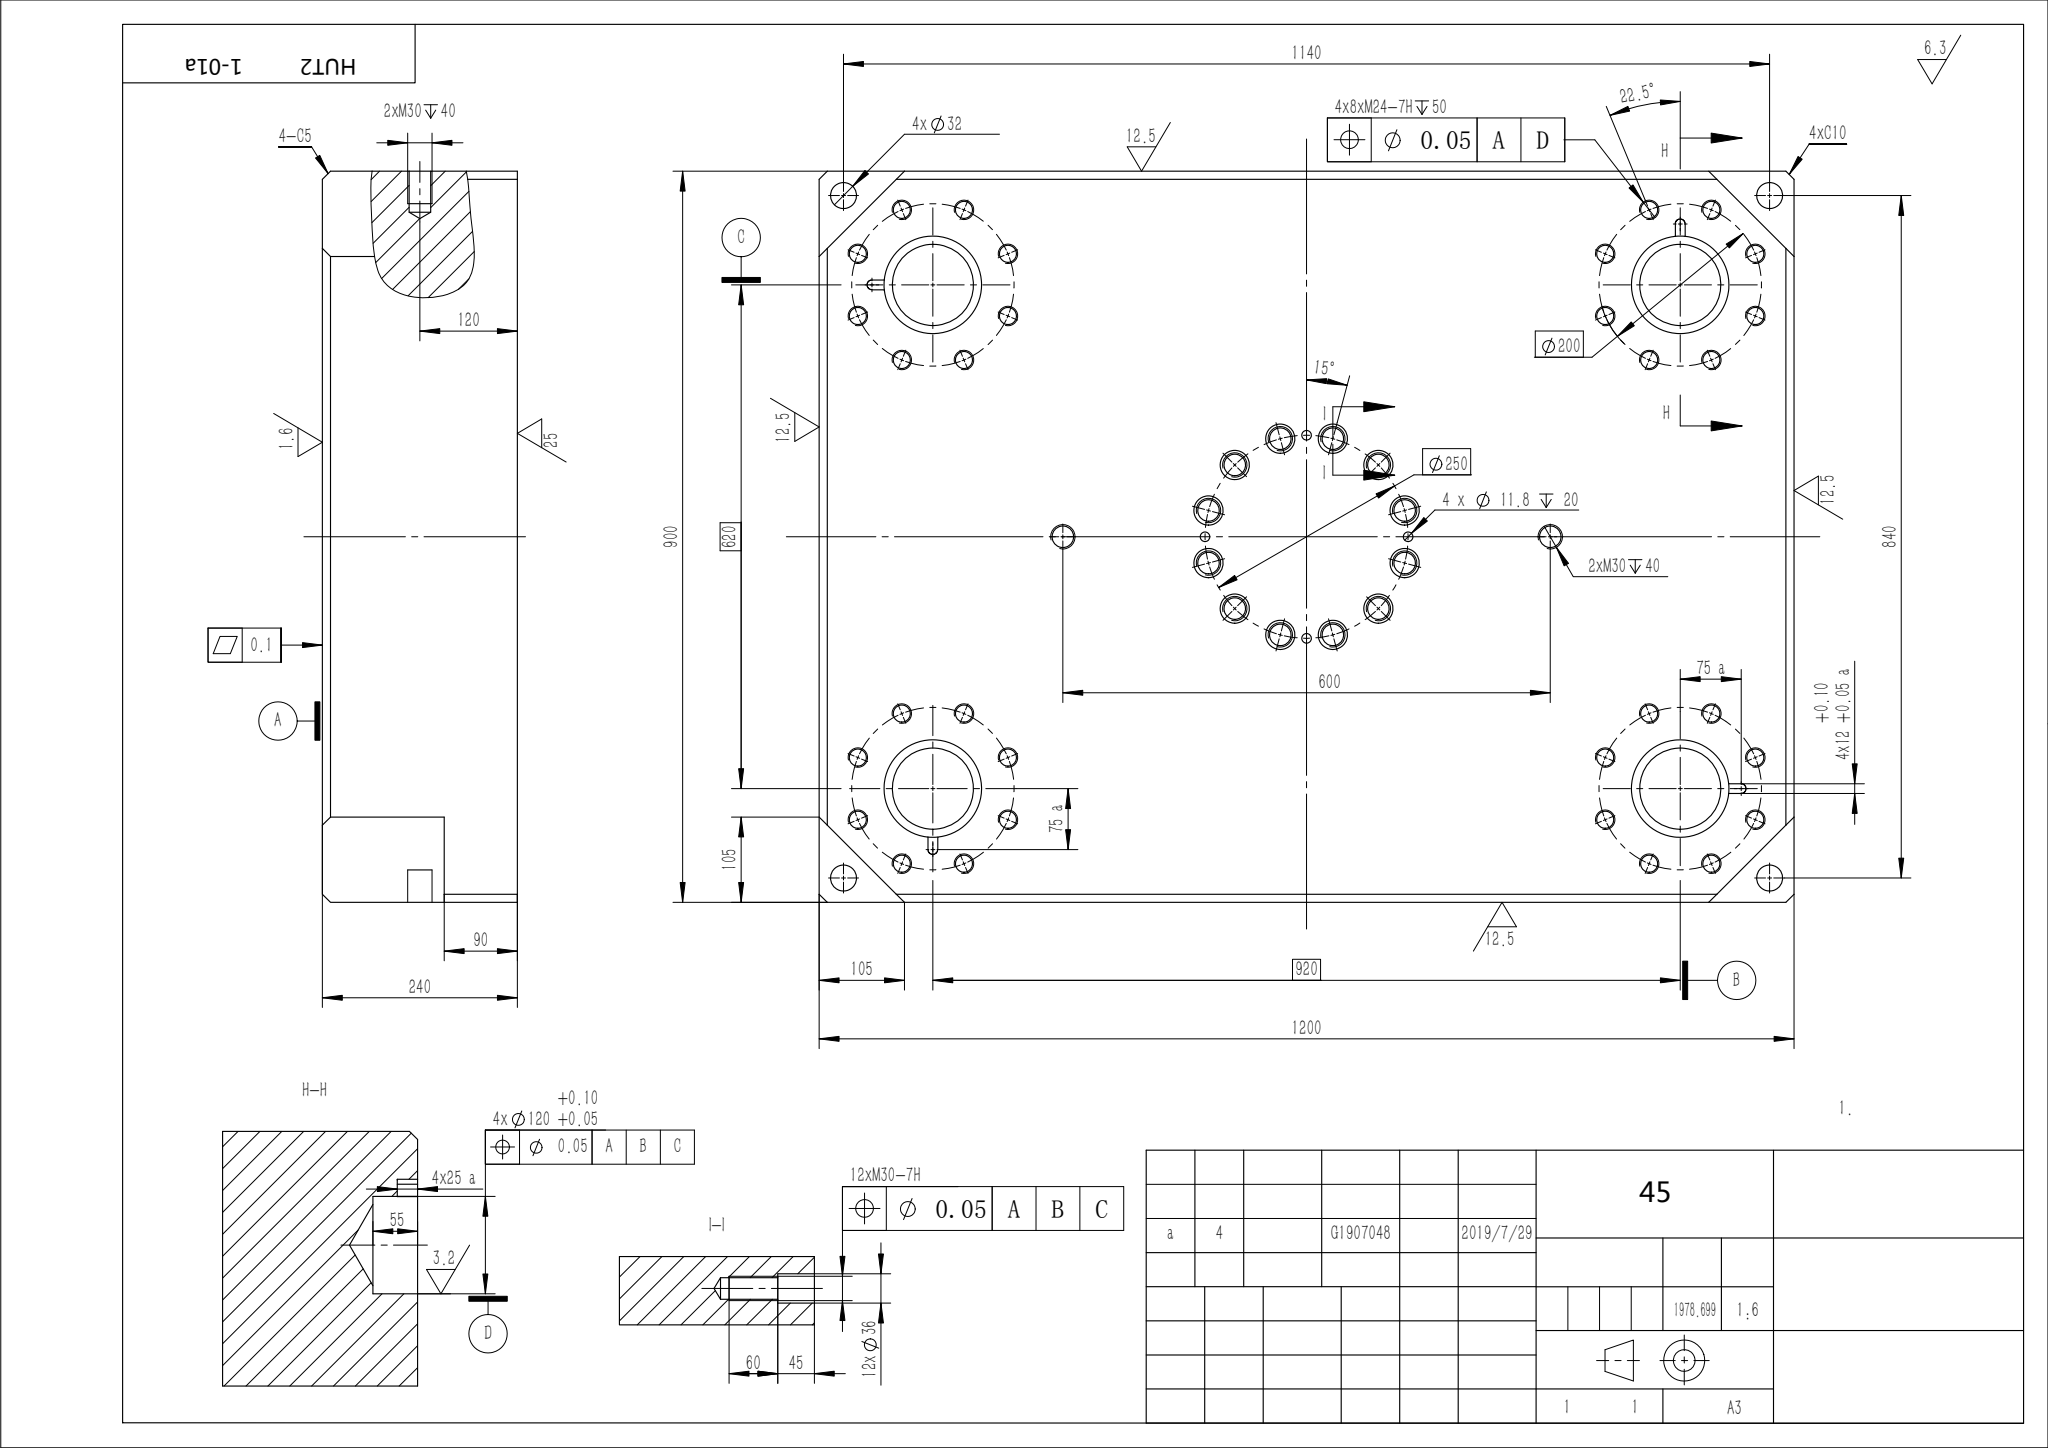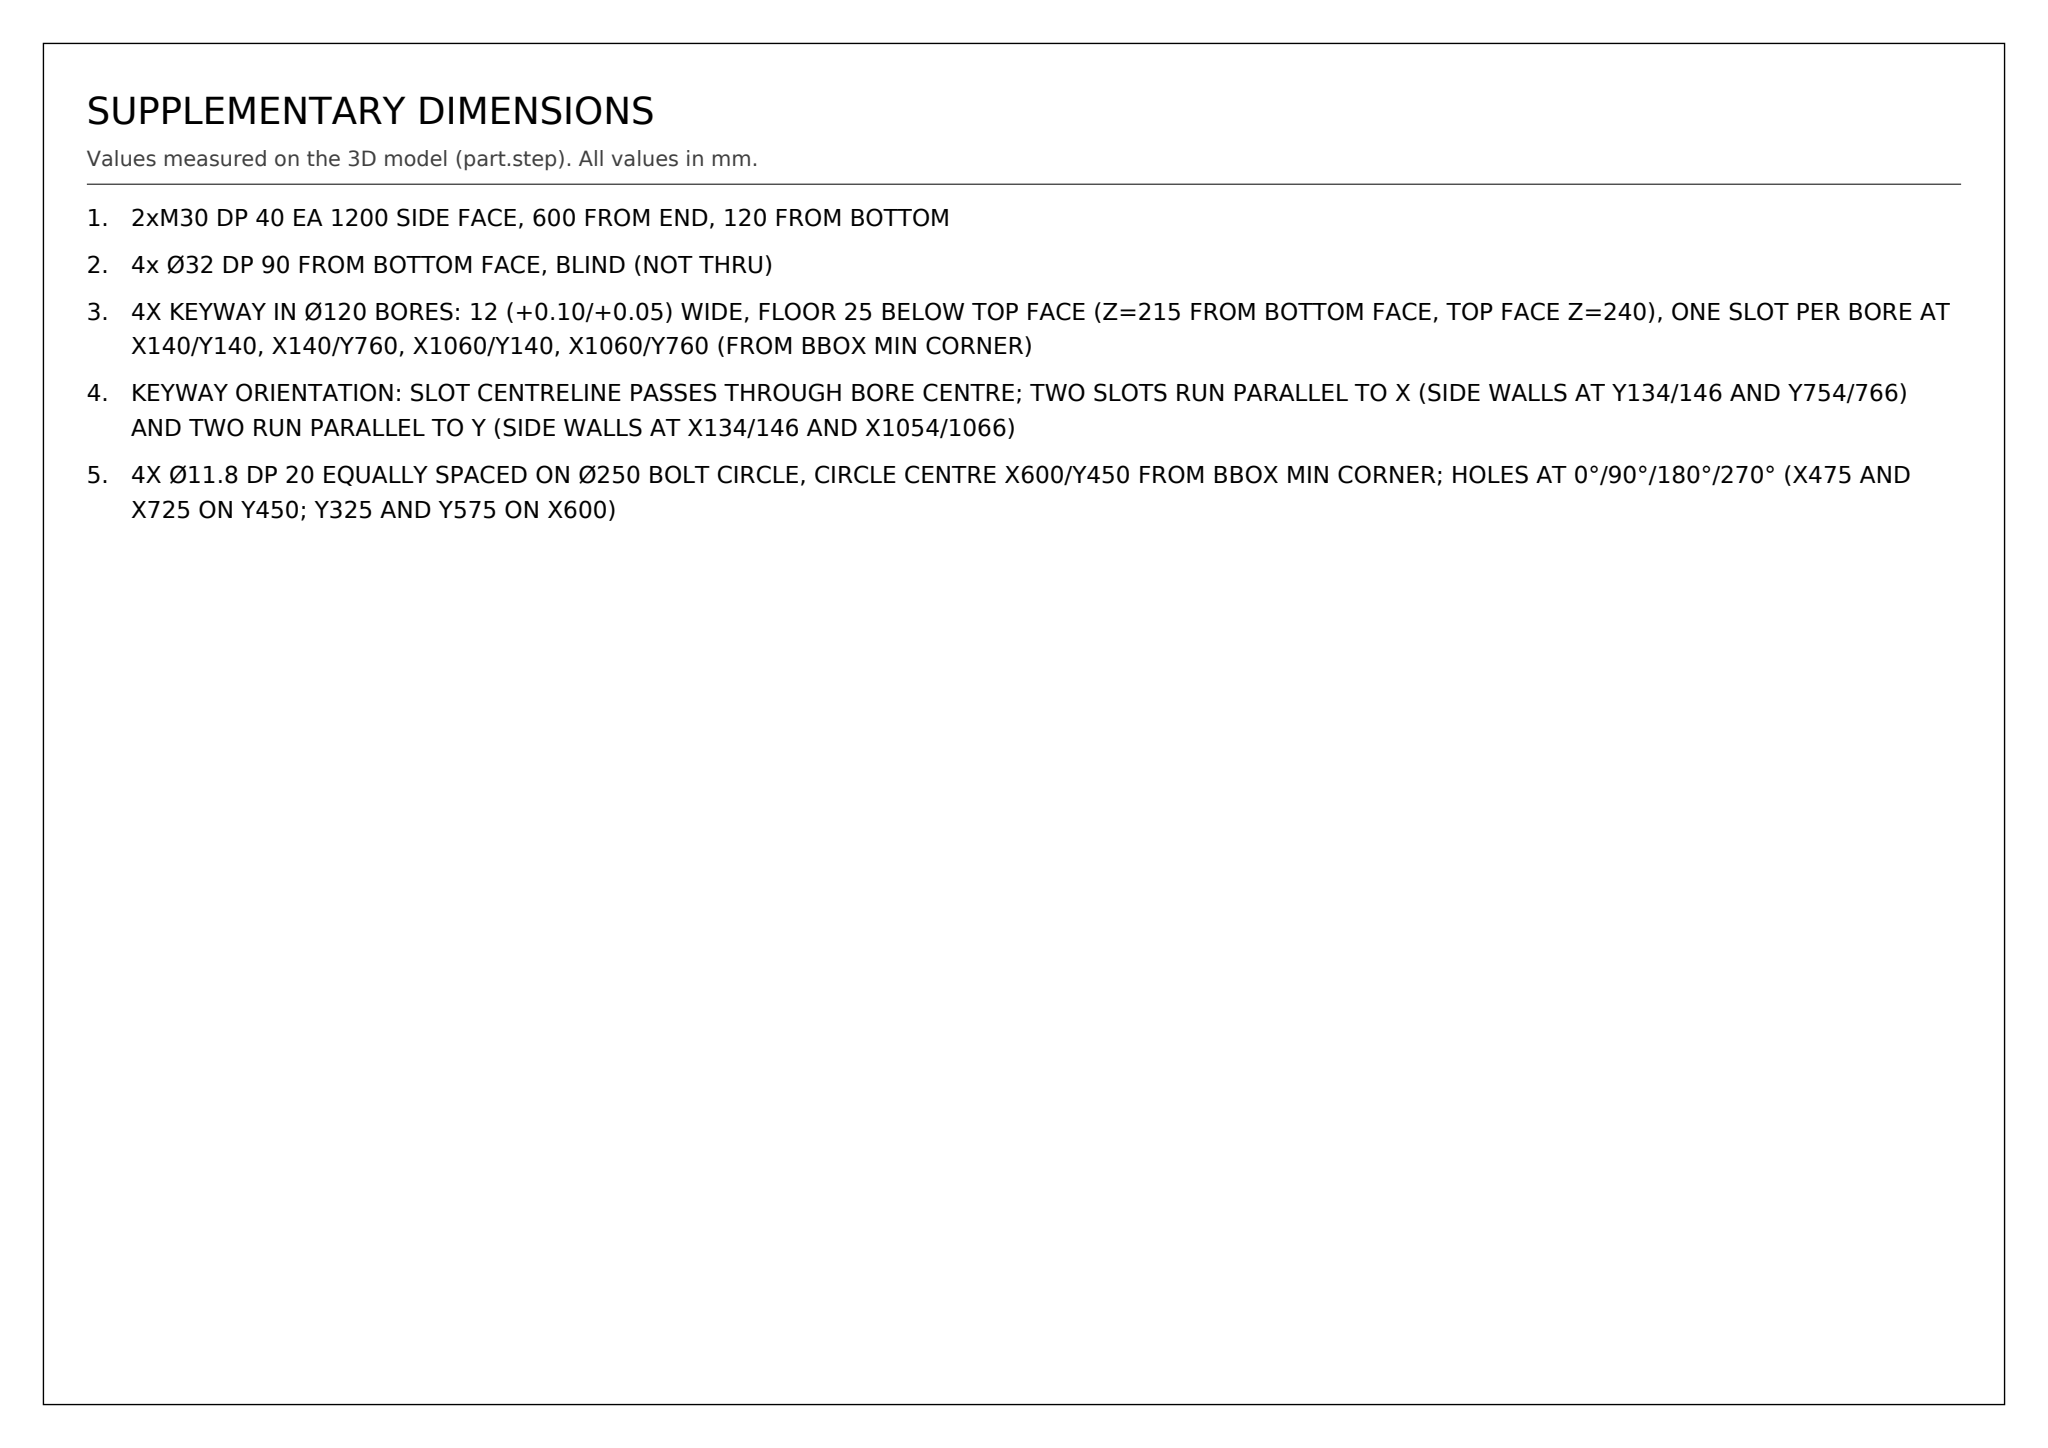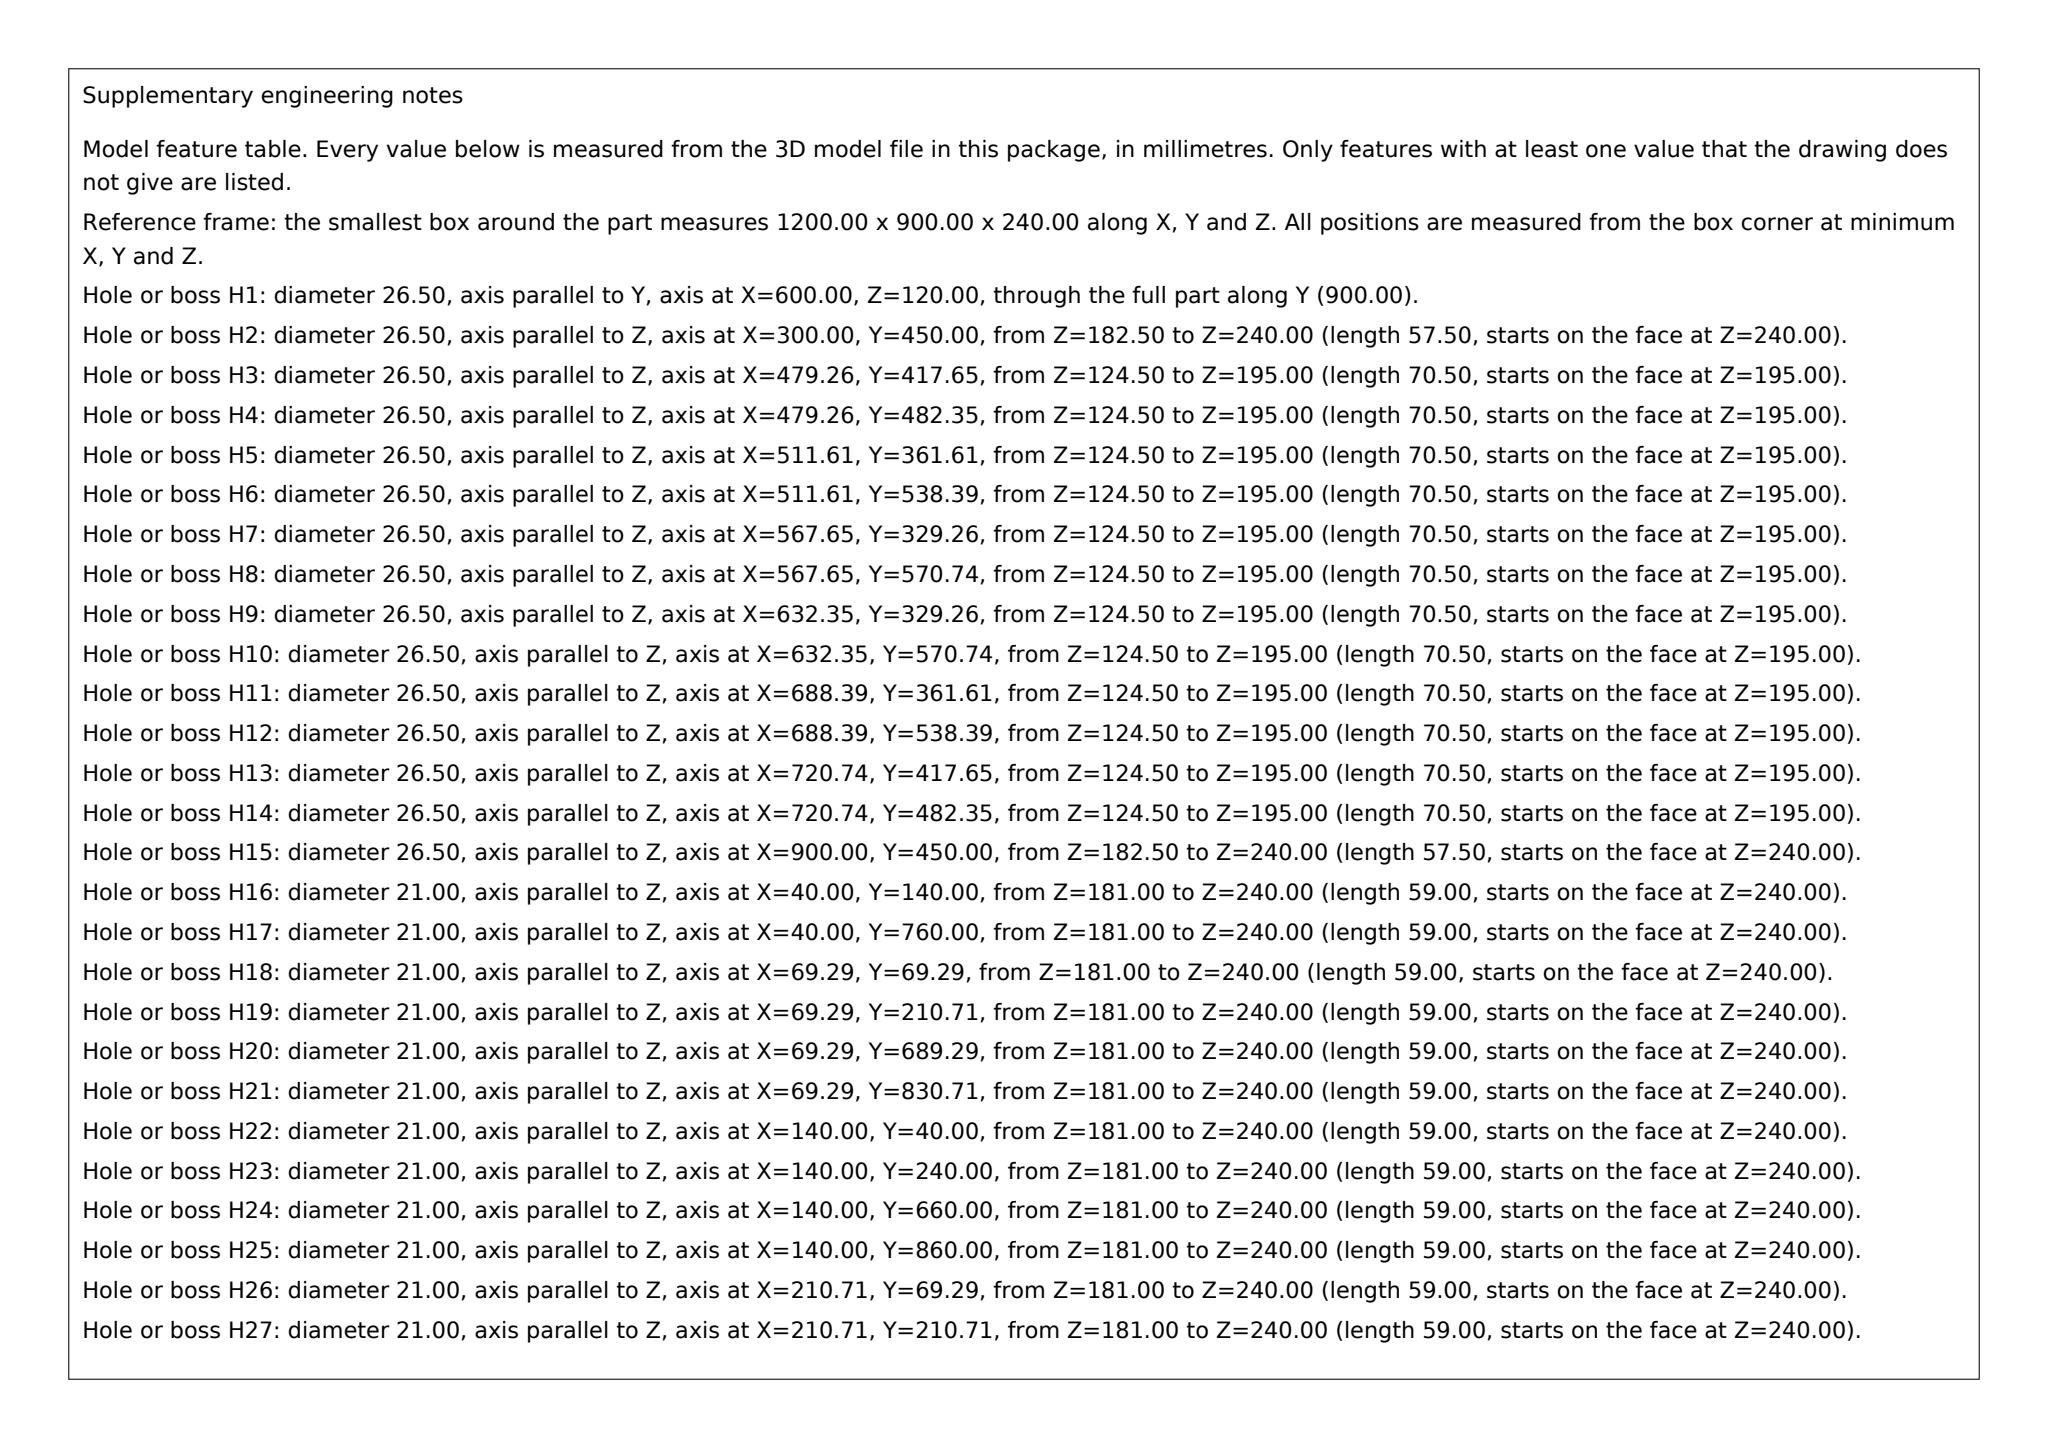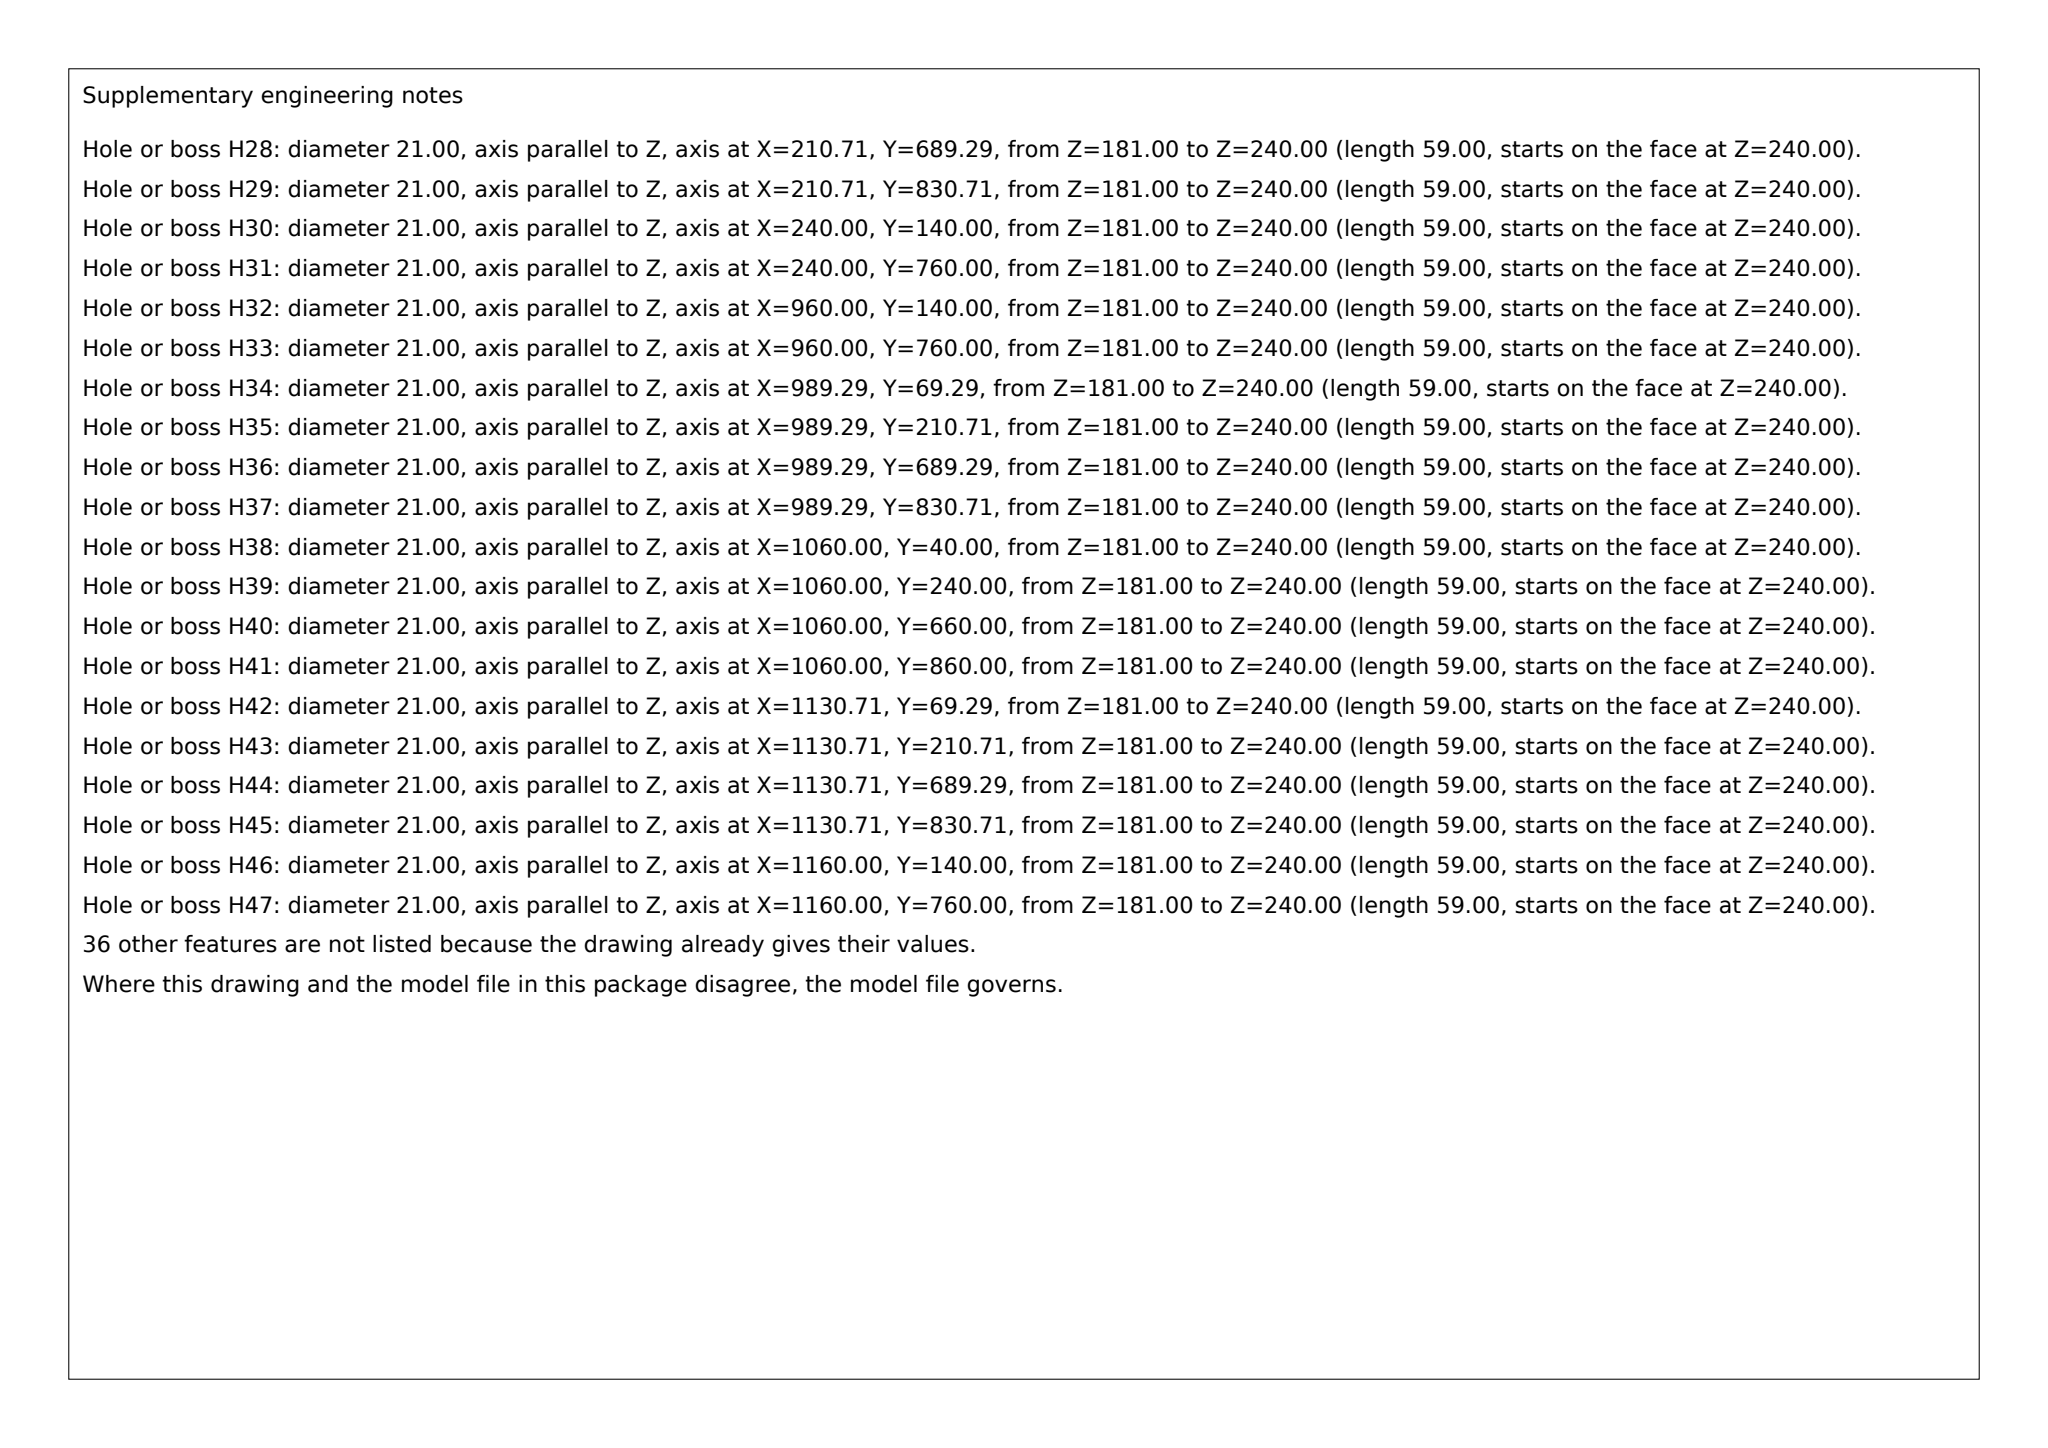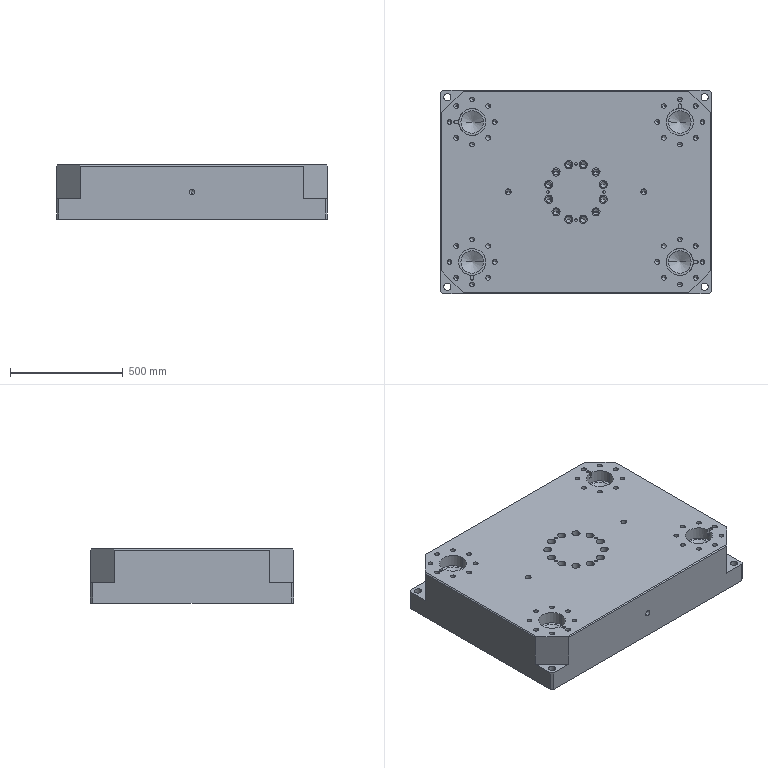Part | SolidWorks | mm | 1 solid | 307 faces | box 1200 x 900 x 240 mm | volume 250876066 mm3 | cylinder 149 | cone 104 | plane 54 | commonest cylinder face diameters 21 x64 26.5 x32 36 x24 11.8 x8 120 x8 32 x8 12 x5
Drawing notes:
2xM30 DP 40 EA 1200 SIDE FACE, 600 FROM END, 120 FROM BOTTOM | from the solid: cyl dia 26.5 axis y at x=600, z=120, len 57.5, count 4 (2 per y=0/y=900 face); M30 thread depth 40 per existing callout
4x Ø32 DP 90 FROM BOTTOM FACE, BLIND (NOT THRU) | from the solid: cylinders dia 32, axis z, length 90.0 at (30,30),(30,870),(1170,30),(1170,870); z-plane at 90.0
4X KEYWAY IN Ø120 BORES: 12 (+0.10/+0.05) WIDE, FLOOR 25 BELOW TOP FACE (Z=215 FROM BOTTOM FACE, TOP FACE Z=240), ONE SLOT PER BORE AT X140/Y140, X140/Y760, X1060/Y140, X1060/Y760 (FROM BBOX MIN CORNER) | from the solid: axis_planes x134/x146, y134/y146, y754/y766, x1054/x1066 (12 apart) with z215 floor planes (count 4); Ø120 z-cylinders at (140,140),(140,760),(1060,140),(1060,760), depth 55
KEYWAY ORIENTATION: SLOT CENTRELINE PASSES THROUGH BORE CENTRE; TWO SLOTS RUN PARALLEL TO X (SIDE WALLS AT Y134/146 AND Y754/766) AND TWO RUN PARALLEL TO Y (SIDE WALLS AT X134/146 AND X1054/1066) | from the solid: axis_planes[x,134]/[x,146], [y,134]/[y,146], [y,754]/[y,766], [x,1054]/[x,1066] each count 1
4X Ø11.8 DP 20 EQUALLY SPACED ON Ø250 BOLT CIRCLE, CIRCLE CENTRE X600/Y450 FROM BBOX MIN CORNER; HOLES AT 0°/90°/180°/270° (X475 AND X725 ON Y450; Y325 AND Y575 ON X600) | from the solid: cylinders[11.8,z] at (475,450),(600,325),(600,575),(725,450), length 20